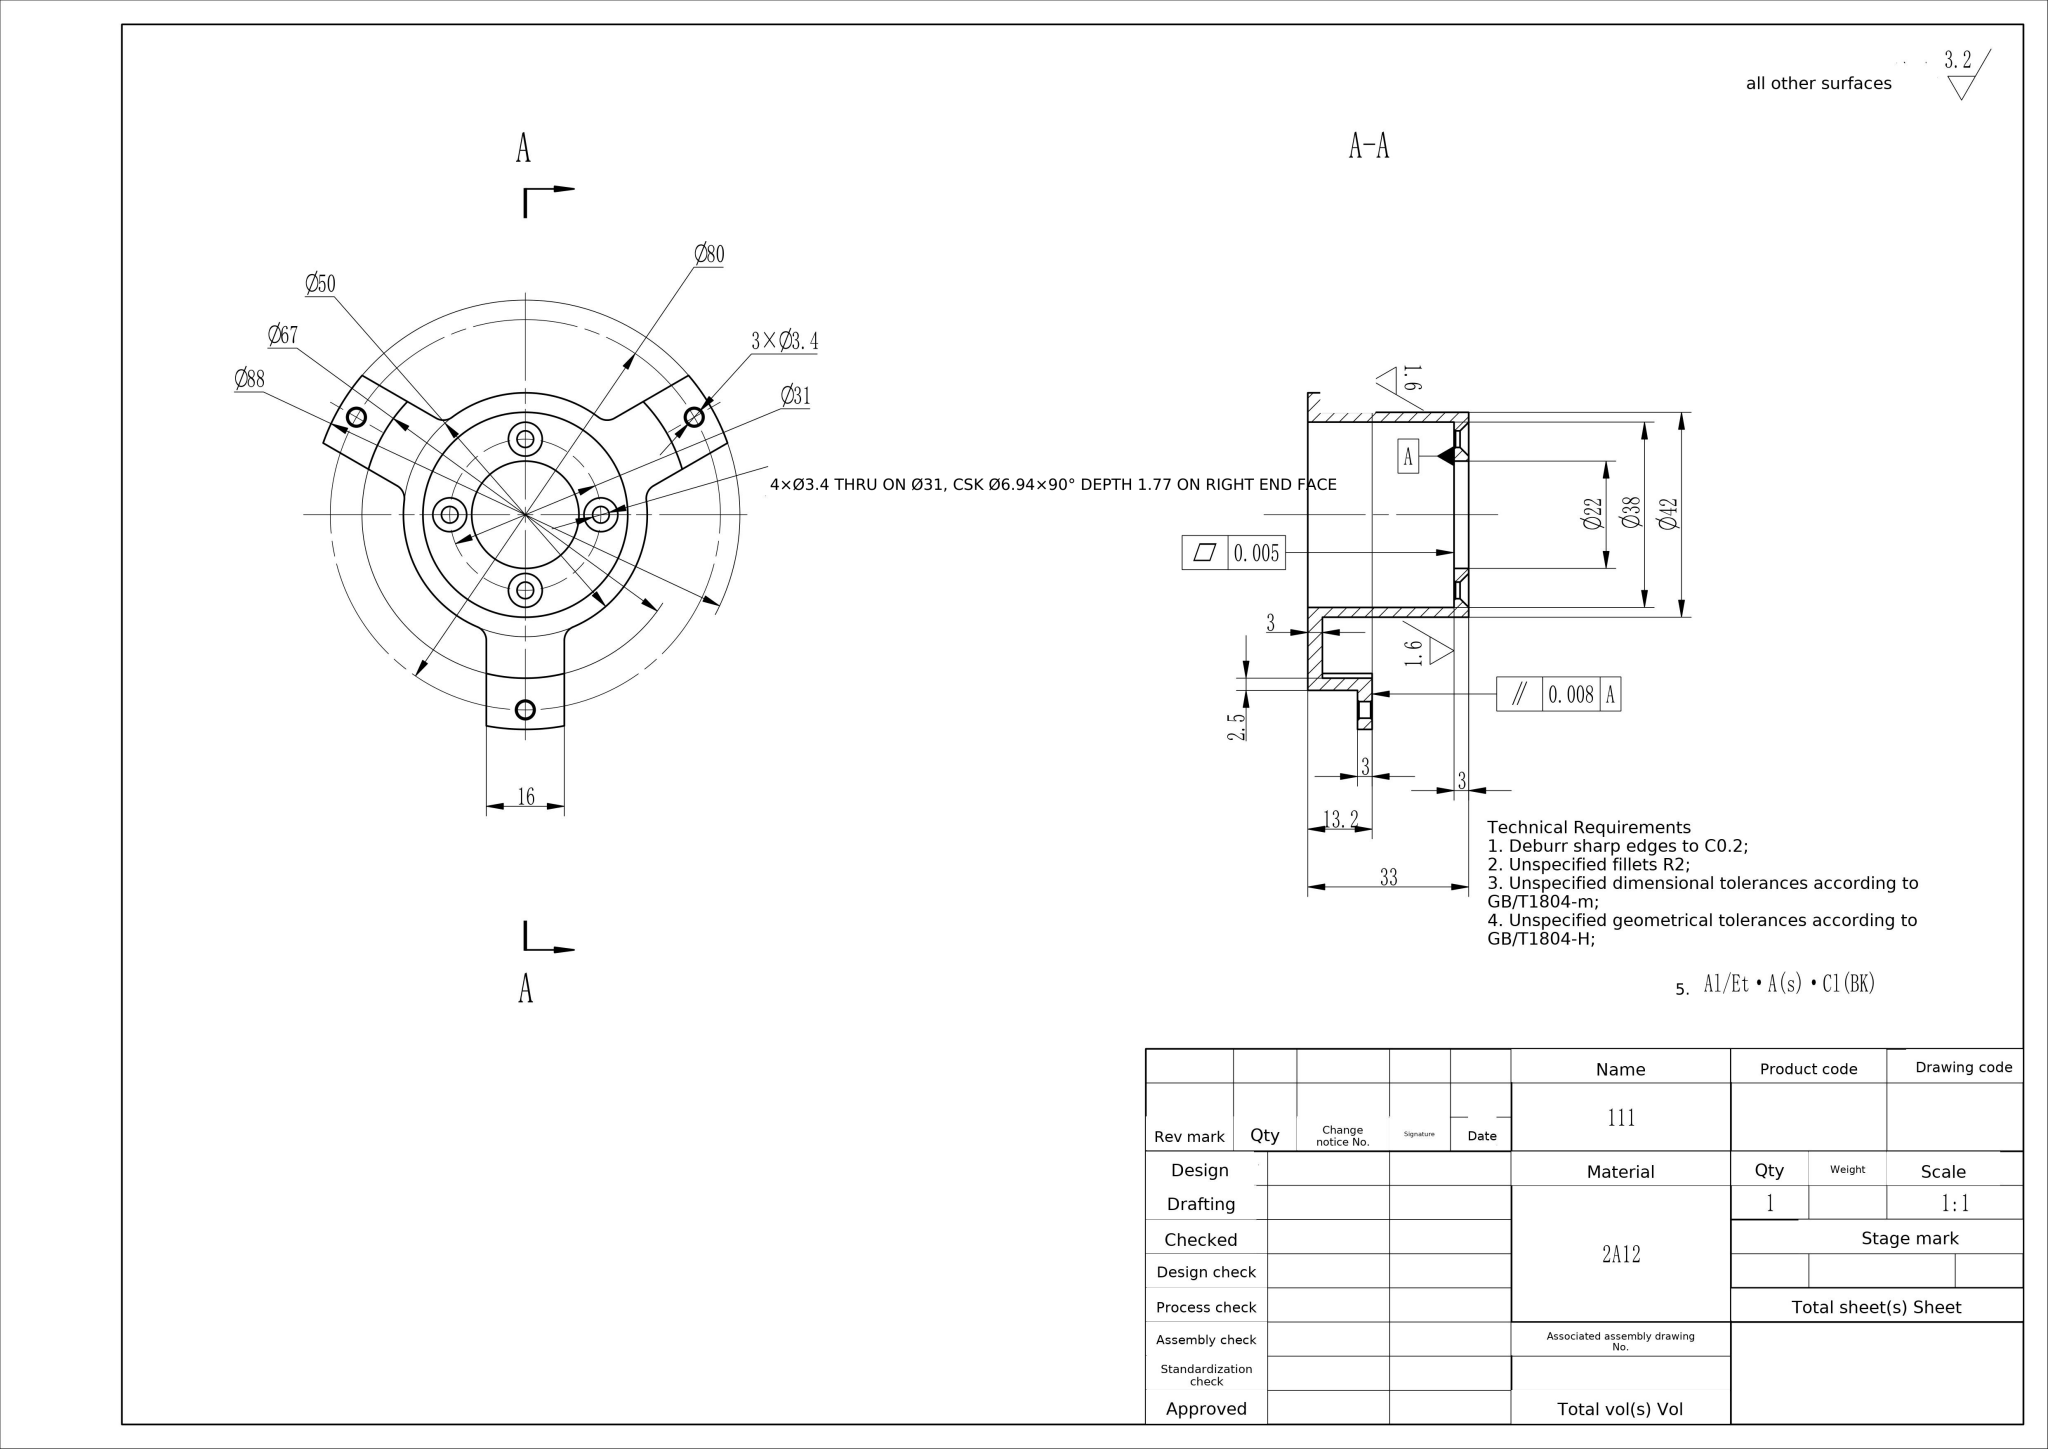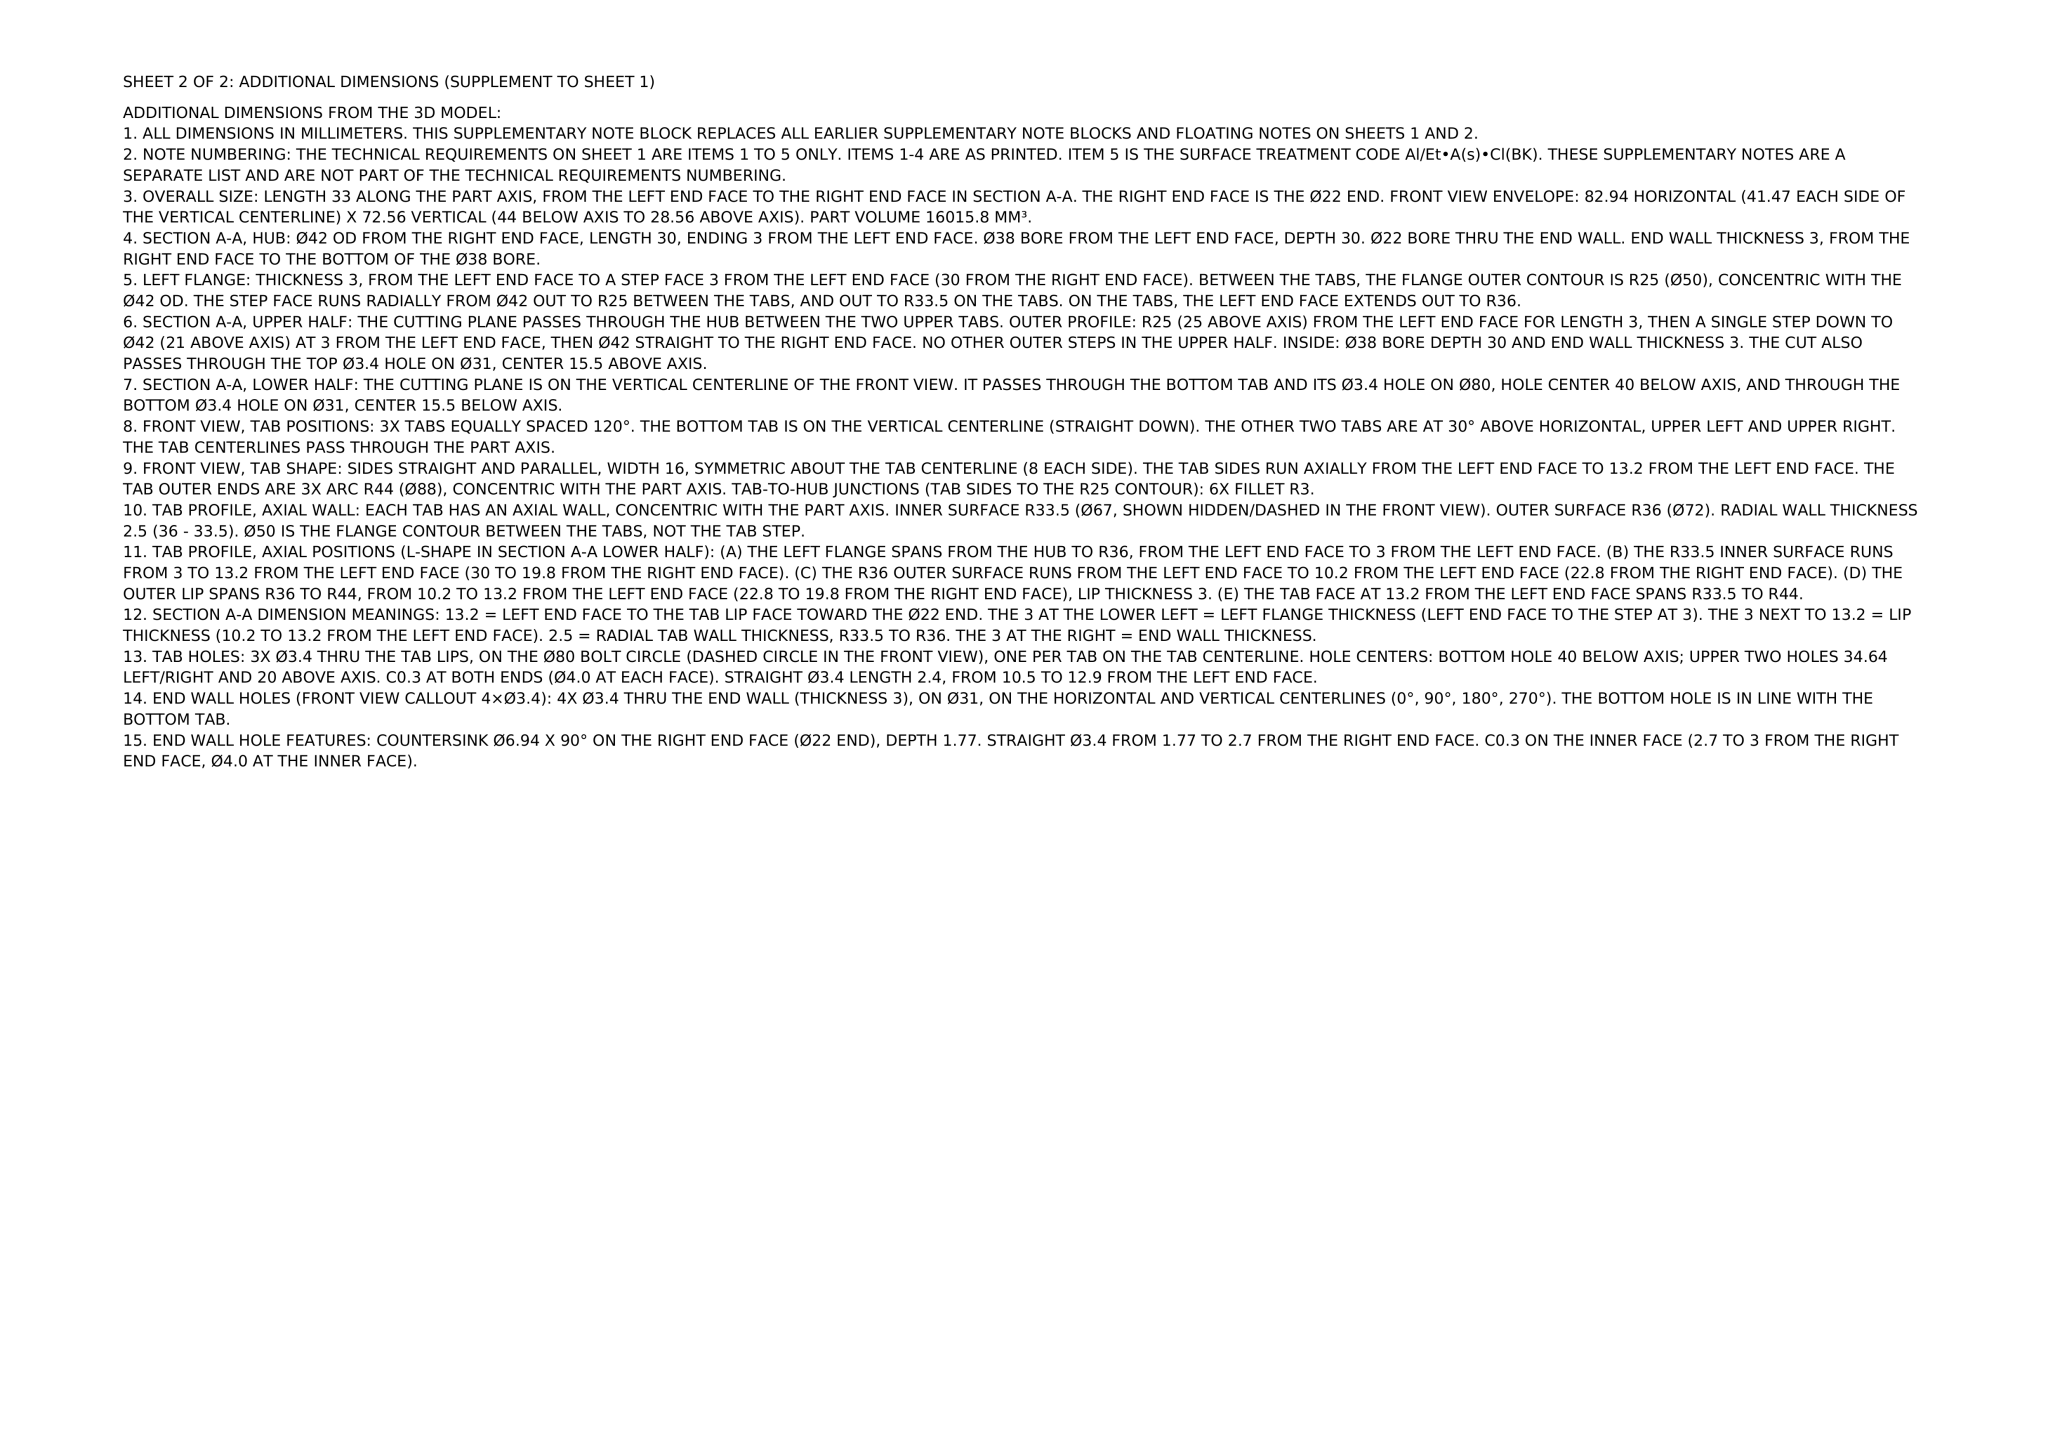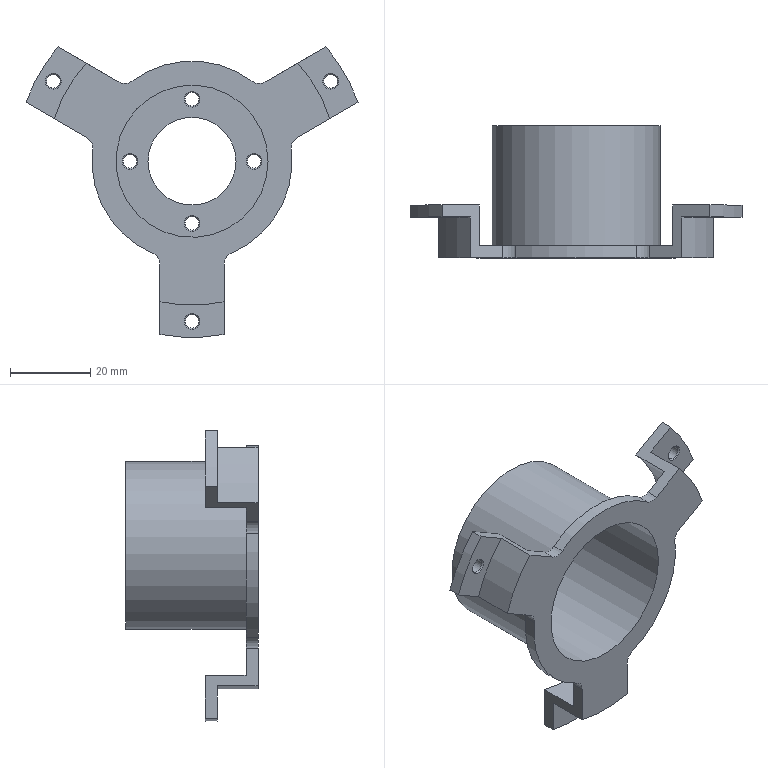Part | NX | mm | 1 solid | 58 faces | box 82.94 x 33 x 72.56 mm | volume 16016 mm3 | cylinder 28 | plane 16 | cone 14 | commonest cylinder face diameters 3.4 x7 6 x6 72 x3 67 x3 88 x3 50 x3 42 x1 22 x1